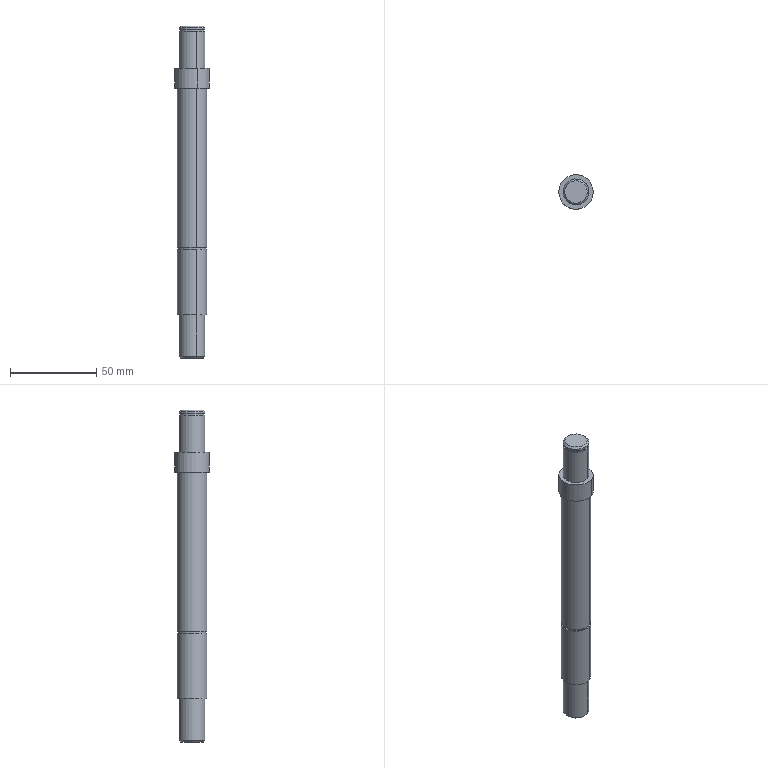Component | SolidWorks | DoubleFilmTransport-1_DriveWheelDriveAxis-2 | 1 solid | 41 faces | box 20 x 20 x 192 mm | volume 41643 mm3 | cylinder 22 | plane 15 | cone 4 | commonest cylinder face diameters 5 x6 15 x6 17 x4 16 x2 20 x2 14 x2
build123d program:
from build123d import *

# Parameters (mm, degrees)
BOSS_EXTRUDE1_START     = 24
SKETCH2_R               = 7.5
BOSS_EXTRUDE1_DEPTH     = 24
SKETCH3_R               = 7.5
BOSS_EXTRUDE2_DEPTH     = 1
BOSS_EXTRUDE2_TAPER     = 45
CUT_EXTRUDE1_REACH      = 194.844
CUT_EXTRUDE1_END_RADIUS = 7.5
CUT_EXTRUDE2_REACH      = 194.844
CUT_EXTRUDE2_END_RADIUS = 7.5


with BuildPart() as part:
    # Sketch1 → Revolve1 (revolve)
    with BuildSketch(Plane.XY):
        Polygon((25, 8.5), (25, 0), (192, 0), (192, 6.5), (191, 7.5), (190.1, 7.5), (190.1, 7), (189, 7), (189, 7.5), (167.5, 7.5), (167.5, 10), (156, 10), (156, 8.5), (64, 8.5), (64, 8), (62.9, 8), (62.9, 8.5), align=None)
    revolve(axis=Axis((25, 0, 0), (1, 0, 0)))

    # Sketch2 → Boss-Extrude1 (add)
    with BuildSketch(Plane.ZY.offset(-25).offset(BOSS_EXTRUDE1_START)):
        with Locations(Location((0, 0, 0), (0, 0, 90))):
            Circle(SKETCH2_R)
    extrude(amount=-BOSS_EXTRUDE1_DEPTH)

    # Sketch3 → Boss-Extrude2 (add)
    with BuildSketch(Plane.ZY.offset(-1)):
        with Locations(Location((0, 0, 0), (0, 0, 90))):
            Circle(SKETCH3_R)
    extrude(amount=BOSS_EXTRUDE2_DEPTH, taper=BOSS_EXTRUDE2_TAPER)

    # Cut-Extrude1: up to this cylinder (the profile starts inside it)
    cut_extrude1_end = Plane(origin=(9, 0, 0), z_dir=(1, 0, 0)) * Cylinder(CUT_EXTRUDE1_END_RADIUS, 405.688, mode=Mode.PRIVATE)
    # Sketch4 → Cut-Extrude1 (cut, up to the surface)
    with BuildSketch(Plane(origin=(0, 0, 5), x_dir=(-1, 0, 0), z_dir=(0, 0, -1)), mode=Mode.PRIVATE) as cut_extrude1_sk1:
        with BuildLine():
            Line((-3.5, 2.5), (-14.5, 2.5))
            ThreePointArc((-14.5, 2.5), (-17, 0), (-14.5, -2.5))
            Line((-14.5, -2.5), (-3.5, -2.5))
            ThreePointArc((-3.5, -2.5), (-1, 0), (-3.5, 2.5))
        make_face()
    cut_extrude1_tool1 = extrude(cut_extrude1_sk1.sketch, amount=-CUT_EXTRUDE1_REACH, mode=Mode.PRIVATE) & cut_extrude1_end
    add(cut_extrude1_tool1.solids().sort_by_distance((9, 0, 5))[0], mode=Mode.SUBTRACT)

    # Cut-Extrude2: up to this cylinder (the profile starts inside it)
    cut_extrude2_end = Plane(origin=(179, 0, 0), z_dir=(1, 0, 0)) * Cylinder(CUT_EXTRUDE2_END_RADIUS, 405.688, mode=Mode.PRIVATE)
    # Sketch5 → Cut-Extrude2 (cut, up to the surface)
    with BuildSketch(Plane(origin=(0, 0, 5), x_dir=(-1, 0, 0), z_dir=(0, 0, -1)), mode=Mode.PRIVATE) as cut_extrude2_sk1:
        with BuildLine():
            Line((-173.5, 2.5), (-184.5, 2.5))
            ThreePointArc((-184.5, 2.5), (-187, 0), (-184.5, -2.5))
            Line((-184.5, -2.5), (-173.5, -2.5))
            ThreePointArc((-173.5, -2.5), (-171, 0), (-173.5, 2.5))
        make_face()
    cut_extrude2_tool1 = extrude(cut_extrude2_sk1.sketch, amount=-CUT_EXTRUDE2_REACH, mode=Mode.PRIVATE) & cut_extrude2_end
    add(cut_extrude2_tool1.solids().sort_by_distance((179, 0, 5))[0], mode=Mode.SUBTRACT)


solid = part.part

# Placed as in the assembly
solid = solid.moved(Location((-212.816, 83.373, -62.5), (-90, 70.831, -90)))